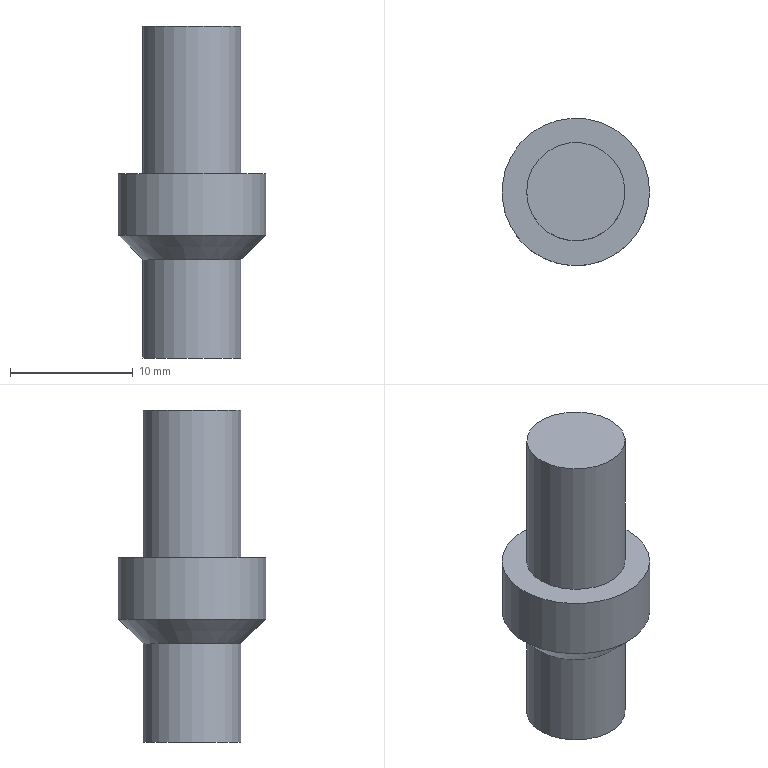Component | NX | PUNCH | 1 solid | 7 faces | box 12 x 12 x 27 mm | volume 1730 mm3 | plane 3 | cylinder 3 | cone 1 | commonest cylinder face diameters 8 x2 12 x1
STEP:
#1=CARTESIAN_POINT('',(0.,0.,0.));
#2=DIRECTION('',(0.,0.,1.));
#3=DIRECTION('',(1.,0.,0.));
#4=AXIS2_PLACEMENT_3D('',#1,#2,#3);
#5=CARTESIAN_POINT('',(11.5,0.,-25.997));
#6=VERTEX_POINT('',#5);
#7=CARTESIAN_POINT('',(7.5,0.,-25.997));
#8=DIRECTION('',(0.,0.,1.));
#9=DIRECTION('',(1.,0.,0.));
#10=AXIS2_PLACEMENT_3D('',#7,#8,#9);
#11=CIRCLE('',#10,4.);
#12=CARTESIAN_POINT('',(7.5,-4.,-25.997));
#13=DIRECTION('',(0.,0.,-1.));
#14=DIRECTION('',(-1.,0.,0.));
#15=AXIS2_PLACEMENT_3D('',#12,#13,#14);
#16=PLANE('',#15);
#17=CARTESIAN_POINT('',(-4.,4.));
#18=CARTESIAN_POINT('',(-4.,10.928));
#19=CARTESIAN_POINT('',(2.,7.464));
#20=CARTESIAN_POINT('',(8.,4.));
#21=CARTESIAN_POINT('',(2.,0.5359));
#22=CARTESIAN_POINT('',(-4.,-2.928));
#23=CARTESIAN_POINT('',(-4.,4.));
#24=(BOUNDED_CURVE()B_SPLINE_CURVE(2,(#17,#18,#19,#20,#21,#22,#23),.UNSPECIFIED.,.T.,.F.)B_SPLINE_CURVE_WITH_KNOTS((1,2,2,2,2,1),(-2.094,0.,2.094,4.189,6.283,8.378),.UNSPECIFIED.)CURVE()GEOMETRIC_REPRESENTATION_ITEM()RATIONAL_B_SPLINE_CURVE((1.,0.5,1.,0.5,1.,0.5,1.))REPRESENTATION_ITEM(''));
#25=(GEOMETRIC_REPRESENTATION_CONTEXT(2)PARAMETRIC_REPRESENTATION_CONTEXT()REPRESENTATION_CONTEXT('',''));
#26=DEFINITIONAL_REPRESENTATION('',(#24),#25);
#27=PCURVE('',#16,#26);
#28=CARTESIAN_POINT('',(7.5,0.,-25.997));
#29=DIRECTION('',(0.,0.,1.));
#30=DIRECTION('',(1.,0.,0.));
#31=AXIS2_PLACEMENT_3D('',#28,#29,#30);
#32=CYLINDRICAL_SURFACE('',#31,4.);
#33=CARTESIAN_POINT('',(0.,0.));
#34=DIRECTION('',(1.,0.));
#35=VECTOR('',#34,1.);
#36=LINE('',#33,#35);
#37=(GEOMETRIC_REPRESENTATION_CONTEXT(2)PARAMETRIC_REPRESENTATION_CONTEXT()REPRESENTATION_CONTEXT('',''));
#38=DEFINITIONAL_REPRESENTATION('',(#36),#37);
#39=PCURVE('',#32,#38);
#40=SURFACE_CURVE('',#11,(#27,#39),.PCURVE_S1.);
#41=EDGE_CURVE('',#6,#6,#40,.T.);
#42=ORIENTED_EDGE('',*,*,#41,.F.);
#43=EDGE_LOOP('',(#42));
#44=FACE_BOUND('',#43,.T.);
#45=ADVANCED_FACE('',(#44),#16,.T.);
#46=ORIENTED_EDGE('',*,*,#41,.T.);
#47=CARTESIAN_POINT('',(11.5,0.,-17.997));
#48=VERTEX_POINT('',#47);
#49=CARTESIAN_POINT('',(11.5,0.,-25.997));
#50=CARTESIAN_POINT('',(11.5,0.,-17.997));
#51=B_SPLINE_CURVE_WITH_KNOTS('',1,(#49,#50),.UNSPECIFIED.,.F.,.F.,(2,2),(0.,8.),.PIECEWISE_BEZIER_KNOTS.);
#52=CARTESIAN_POINT('',(6.283,0.));
#53=DIRECTION('',(0.,1.));
#54=VECTOR('',#53,1.);
#55=LINE('',#52,#54);
#56=(GEOMETRIC_REPRESENTATION_CONTEXT(2)PARAMETRIC_REPRESENTATION_CONTEXT()REPRESENTATION_CONTEXT('',''));
#57=DEFINITIONAL_REPRESENTATION('',(#55),#56);
#58=PCURVE('',#32,#57);
#59=CARTESIAN_POINT('',(0.,0.));
#60=DIRECTION('',(0.,1.));
#61=VECTOR('',#60,1.);
#62=LINE('',#59,#61);
#63=(GEOMETRIC_REPRESENTATION_CONTEXT(2)PARAMETRIC_REPRESENTATION_CONTEXT()REPRESENTATION_CONTEXT('',''));
#64=DEFINITIONAL_REPRESENTATION('',(#62),#63);
#65=PCURVE('',#32,#64);
#66=SEAM_CURVE('',#51,(#58,#65),.PCURVE_S1.);
#67=EDGE_CURVE('',#6,#48,#66,.T.);
#68=ORIENTED_EDGE('',*,*,#67,.T.);
#69=CARTESIAN_POINT('',(7.5,0.,-17.997));
#70=DIRECTION('',(0.,0.,1.));
#71=DIRECTION('',(1.,0.,0.));
#72=AXIS2_PLACEMENT_3D('',#69,#70,#71);
#73=CIRCLE('',#72,4.);
#74=CARTESIAN_POINT('',(0.,8.));
#75=DIRECTION('',(1.,0.));
#76=VECTOR('',#75,1.);
#77=LINE('',#74,#76);
#78=(GEOMETRIC_REPRESENTATION_CONTEXT(2)PARAMETRIC_REPRESENTATION_CONTEXT()REPRESENTATION_CONTEXT('',''));
#79=DEFINITIONAL_REPRESENTATION('',(#77),#78);
#80=PCURVE('',#32,#79);
#81=CARTESIAN_POINT('',(7.5,0.,-15.997));
#82=DIRECTION('',(0.,0.,1.));
#83=DIRECTION('',(1.,0.,0.));
#84=AXIS2_PLACEMENT_3D('',#81,#82,#83);
#85=CONICAL_SURFACE('',#84,6.,0.7854);
#86=CARTESIAN_POINT('',(0.,-2.));
#87=DIRECTION('',(1.,0.));
#88=VECTOR('',#87,1.);
#89=LINE('',#86,#88);
#90=(GEOMETRIC_REPRESENTATION_CONTEXT(2)PARAMETRIC_REPRESENTATION_CONTEXT()REPRESENTATION_CONTEXT('',''));
#91=DEFINITIONAL_REPRESENTATION('',(#89),#90);
#92=PCURVE('',#85,#91);
#93=SURFACE_CURVE('',#73,(#80,#92),.PCURVE_S1.);
#94=EDGE_CURVE('',#48,#48,#93,.T.);
#95=ORIENTED_EDGE('',*,*,#94,.F.);
#96=ORIENTED_EDGE('',*,*,#67,.F.);
#97=EDGE_LOOP('',(#46,#68,#95,#96));
#98=FACE_BOUND('',#97,.T.);
#99=ADVANCED_FACE('',(#98),#32,.T.);
#100=ORIENTED_EDGE('',*,*,#94,.T.);
#101=CARTESIAN_POINT('',(13.5,0.,-15.997));
#102=VERTEX_POINT('',#101);
#103=CARTESIAN_POINT('',(11.5,0.,-17.997));
#104=CARTESIAN_POINT('',(13.5,0.,-15.997));
#105=B_SPLINE_CURVE_WITH_KNOTS('',1,(#103,#104),.UNSPECIFIED.,.F.,.F.,(2,2),(-2.828,0.),.PIECEWISE_BEZIER_KNOTS.);
#106=CARTESIAN_POINT('',(6.283,0.));
#107=DIRECTION('',(0.,1.));
#108=VECTOR('',#107,1.);
#109=LINE('',#106,#108);
#110=(GEOMETRIC_REPRESENTATION_CONTEXT(2)PARAMETRIC_REPRESENTATION_CONTEXT()REPRESENTATION_CONTEXT('',''));
#111=DEFINITIONAL_REPRESENTATION('',(#109),#110);
#112=PCURVE('',#85,#111);
#113=CARTESIAN_POINT('',(0.,0.));
#114=DIRECTION('',(0.,1.));
#115=VECTOR('',#114,1.);
#116=LINE('',#113,#115);
#117=(GEOMETRIC_REPRESENTATION_CONTEXT(2)PARAMETRIC_REPRESENTATION_CONTEXT()REPRESENTATION_CONTEXT('',''));
#118=DEFINITIONAL_REPRESENTATION('',(#116),#117);
#119=PCURVE('',#85,#118);
#120=SEAM_CURVE('',#105,(#112,#119),.PCURVE_S1.);
#121=EDGE_CURVE('',#48,#102,#120,.T.);
#122=ORIENTED_EDGE('',*,*,#121,.T.);
#123=CARTESIAN_POINT('',(7.5,0.,-15.997));
#124=DIRECTION('',(0.,0.,1.));
#125=DIRECTION('',(1.,0.,0.));
#126=AXIS2_PLACEMENT_3D('',#123,#124,#125);
#127=CIRCLE('',#126,6.);
#128=CARTESIAN_POINT('',(0.,0.));
#129=DIRECTION('',(1.,0.));
#130=VECTOR('',#129,1.);
#131=LINE('',#128,#130);
#132=(GEOMETRIC_REPRESENTATION_CONTEXT(2)PARAMETRIC_REPRESENTATION_CONTEXT()REPRESENTATION_CONTEXT('',''));
#133=DEFINITIONAL_REPRESENTATION('',(#131),#132);
#134=PCURVE('',#85,#133);
#135=CARTESIAN_POINT('',(7.5,0.,-25.997));
#136=DIRECTION('',(0.,0.,1.));
#137=DIRECTION('',(1.,0.,0.));
#138=AXIS2_PLACEMENT_3D('',#135,#136,#137);
#139=CYLINDRICAL_SURFACE('',#138,6.);
#140=CARTESIAN_POINT('',(0.,10.));
#141=DIRECTION('',(1.,0.));
#142=VECTOR('',#141,1.);
#143=LINE('',#140,#142);
#144=(GEOMETRIC_REPRESENTATION_CONTEXT(2)PARAMETRIC_REPRESENTATION_CONTEXT()REPRESENTATION_CONTEXT('',''));
#145=DEFINITIONAL_REPRESENTATION('',(#143),#144);
#146=PCURVE('',#139,#145);
#147=SURFACE_CURVE('',#127,(#134,#146),.PCURVE_S1.);
#148=EDGE_CURVE('',#102,#102,#147,.T.);
#149=ORIENTED_EDGE('',*,*,#148,.F.);
#150=ORIENTED_EDGE('',*,*,#121,.F.);
#151=EDGE_LOOP('',(#100,#122,#149,#150));
#152=FACE_BOUND('',#151,.T.);
#153=ADVANCED_FACE('',(#152),#85,.T.);
#154=ORIENTED_EDGE('',*,*,#148,.T.);
#155=CARTESIAN_POINT('',(13.5,0.,-10.997));
#156=VERTEX_POINT('',#155);
#157=CARTESIAN_POINT('',(13.5,0.,-15.997));
#158=CARTESIAN_POINT('',(13.5,0.,-10.997));
#159=B_SPLINE_CURVE_WITH_KNOTS('',1,(#157,#158),.UNSPECIFIED.,.F.,.F.,(2,2),(10.,15.),.PIECEWISE_BEZIER_KNOTS.);
#160=CARTESIAN_POINT('',(6.283,0.));
#161=DIRECTION('',(0.,1.));
#162=VECTOR('',#161,1.);
#163=LINE('',#160,#162);
#164=(GEOMETRIC_REPRESENTATION_CONTEXT(2)PARAMETRIC_REPRESENTATION_CONTEXT()REPRESENTATION_CONTEXT('',''));
#165=DEFINITIONAL_REPRESENTATION('',(#163),#164);
#166=PCURVE('',#139,#165);
#167=CARTESIAN_POINT('',(0.,0.));
#168=DIRECTION('',(0.,1.));
#169=VECTOR('',#168,1.);
#170=LINE('',#167,#169);
#171=(GEOMETRIC_REPRESENTATION_CONTEXT(2)PARAMETRIC_REPRESENTATION_CONTEXT()REPRESENTATION_CONTEXT('',''));
#172=DEFINITIONAL_REPRESENTATION('',(#170),#171);
#173=PCURVE('',#139,#172);
#174=SEAM_CURVE('',#159,(#166,#173),.PCURVE_S1.);
#175=EDGE_CURVE('',#102,#156,#174,.T.);
#176=ORIENTED_EDGE('',*,*,#175,.T.);
#177=CARTESIAN_POINT('',(7.5,0.,-10.997));
#178=DIRECTION('',(0.,0.,1.));
#179=DIRECTION('',(1.,0.,0.));
#180=AXIS2_PLACEMENT_3D('',#177,#178,#179);
#181=CIRCLE('',#180,6.);
#182=CARTESIAN_POINT('',(0.,15.));
#183=DIRECTION('',(1.,0.));
#184=VECTOR('',#183,1.);
#185=LINE('',#182,#184);
#186=(GEOMETRIC_REPRESENTATION_CONTEXT(2)PARAMETRIC_REPRESENTATION_CONTEXT()REPRESENTATION_CONTEXT('',''));
#187=DEFINITIONAL_REPRESENTATION('',(#185),#186);
#188=PCURVE('',#139,#187);
#189=CARTESIAN_POINT('',(7.5,-4.,-10.997));
#190=DIRECTION('',(0.,0.,1.));
#191=DIRECTION('',(1.,0.,0.));
#192=AXIS2_PLACEMENT_3D('',#189,#190,#191);
#193=PLANE('',#192);
#194=CARTESIAN_POINT('',(0.,4.));
#195=DIRECTION('',(1.,0.));
#196=AXIS2_PLACEMENT_2D('',#194,#195);
#197=CIRCLE('',#196,6.);
#198=(GEOMETRIC_REPRESENTATION_CONTEXT(2)PARAMETRIC_REPRESENTATION_CONTEXT()REPRESENTATION_CONTEXT('',''));
#199=DEFINITIONAL_REPRESENTATION('',(#197),#198);
#200=PCURVE('',#193,#199);
#201=SURFACE_CURVE('',#181,(#188,#200),.PCURVE_S1.);
#202=EDGE_CURVE('',#156,#156,#201,.T.);
#203=ORIENTED_EDGE('',*,*,#202,.F.);
#204=ORIENTED_EDGE('',*,*,#175,.F.);
#205=EDGE_LOOP('',(#154,#176,#203,#204));
#206=FACE_BOUND('',#205,.T.);
#207=ADVANCED_FACE('',(#206),#139,.T.);
#208=ORIENTED_EDGE('',*,*,#202,.T.);
#209=EDGE_LOOP('',(#208));
#210=FACE_BOUND('',#209,.T.);
#211=CARTESIAN_POINT('',(11.5,0.,-10.997));
#212=VERTEX_POINT('',#211);
#213=CARTESIAN_POINT('',(7.5,0.,-10.997));
#214=DIRECTION('',(0.,0.,1.));
#215=DIRECTION('',(1.,0.,0.));
#216=AXIS2_PLACEMENT_3D('',#213,#214,#215);
#217=CIRCLE('',#216,4.);
#218=CARTESIAN_POINT('',(0.,4.));
#219=DIRECTION('',(1.,0.));
#220=AXIS2_PLACEMENT_2D('',#218,#219);
#221=CIRCLE('',#220,4.);
#222=(GEOMETRIC_REPRESENTATION_CONTEXT(2)PARAMETRIC_REPRESENTATION_CONTEXT()REPRESENTATION_CONTEXT('',''));
#223=DEFINITIONAL_REPRESENTATION('',(#221),#222);
#224=PCURVE('',#193,#223);
#225=CARTESIAN_POINT('',(7.5,0.,-25.997));
#226=DIRECTION('',(0.,0.,1.));
#227=DIRECTION('',(1.,0.,0.));
#228=AXIS2_PLACEMENT_3D('',#225,#226,#227);
#229=CYLINDRICAL_SURFACE('',#228,4.);
#230=CARTESIAN_POINT('',(0.,15.));
#231=DIRECTION('',(1.,0.));
#232=VECTOR('',#231,1.);
#233=LINE('',#230,#232);
#234=(GEOMETRIC_REPRESENTATION_CONTEXT(2)PARAMETRIC_REPRESENTATION_CONTEXT()REPRESENTATION_CONTEXT('',''));
#235=DEFINITIONAL_REPRESENTATION('',(#233),#234);
#236=PCURVE('',#229,#235);
#237=SURFACE_CURVE('',#217,(#224,#236),.PCURVE_S1.);
#238=EDGE_CURVE('',#212,#212,#237,.T.);
#239=ORIENTED_EDGE('',*,*,#238,.F.);
#240=EDGE_LOOP('',(#239));
#241=FACE_BOUND('',#240,.T.);
#242=ADVANCED_FACE('',(#210,#241),#193,.T.);
#243=ORIENTED_EDGE('',*,*,#238,.T.);
#244=CARTESIAN_POINT('',(11.5,0.,1.003));
#245=VERTEX_POINT('',#244);
#246=CARTESIAN_POINT('',(11.5,0.,-10.997));
#247=CARTESIAN_POINT('',(11.5,0.,1.003));
#248=B_SPLINE_CURVE_WITH_KNOTS('',1,(#246,#247),.UNSPECIFIED.,.F.,.F.,(2,2),(15.,27.),.PIECEWISE_BEZIER_KNOTS.);
#249=CARTESIAN_POINT('',(6.283,0.));
#250=DIRECTION('',(0.,1.));
#251=VECTOR('',#250,1.);
#252=LINE('',#249,#251);
#253=(GEOMETRIC_REPRESENTATION_CONTEXT(2)PARAMETRIC_REPRESENTATION_CONTEXT()REPRESENTATION_CONTEXT('',''));
#254=DEFINITIONAL_REPRESENTATION('',(#252),#253);
#255=PCURVE('',#229,#254);
#256=CARTESIAN_POINT('',(0.,0.));
#257=DIRECTION('',(0.,1.));
#258=VECTOR('',#257,1.);
#259=LINE('',#256,#258);
#260=(GEOMETRIC_REPRESENTATION_CONTEXT(2)PARAMETRIC_REPRESENTATION_CONTEXT()REPRESENTATION_CONTEXT('',''));
#261=DEFINITIONAL_REPRESENTATION('',(#259),#260);
#262=PCURVE('',#229,#261);
#263=SEAM_CURVE('',#248,(#255,#262),.PCURVE_S1.);
#264=EDGE_CURVE('',#212,#245,#263,.T.);
#265=ORIENTED_EDGE('',*,*,#264,.T.);
#266=CARTESIAN_POINT('',(7.5,0.,1.003));
#267=DIRECTION('',(0.,0.,1.));
#268=DIRECTION('',(1.,0.,0.));
#269=AXIS2_PLACEMENT_3D('',#266,#267,#268);
#270=CIRCLE('',#269,4.);
#271=CARTESIAN_POINT('',(0.,27.));
#272=DIRECTION('',(1.,0.));
#273=VECTOR('',#272,1.);
#274=LINE('',#271,#273);
#275=(GEOMETRIC_REPRESENTATION_CONTEXT(2)PARAMETRIC_REPRESENTATION_CONTEXT()REPRESENTATION_CONTEXT('',''));
#276=DEFINITIONAL_REPRESENTATION('',(#274),#275);
#277=PCURVE('',#229,#276);
#278=CARTESIAN_POINT('',(7.5,0.,1.003));
#279=DIRECTION('',(0.,0.,1.));
#280=DIRECTION('',(1.,0.,0.));
#281=AXIS2_PLACEMENT_3D('',#278,#279,#280);
#282=PLANE('',#281);
#283=CARTESIAN_POINT('',(0.,0.));
#284=DIRECTION('',(1.,0.));
#285=AXIS2_PLACEMENT_2D('',#283,#284);
#286=CIRCLE('',#285,4.);
#287=(GEOMETRIC_REPRESENTATION_CONTEXT(2)PARAMETRIC_REPRESENTATION_CONTEXT()REPRESENTATION_CONTEXT('',''));
#288=DEFINITIONAL_REPRESENTATION('',(#286),#287);
#289=PCURVE('',#282,#288);
#290=SURFACE_CURVE('',#270,(#277,#289),.PCURVE_S1.);
#291=EDGE_CURVE('',#245,#245,#290,.T.);
#292=ORIENTED_EDGE('',*,*,#291,.F.);
#293=ORIENTED_EDGE('',*,*,#264,.F.);
#294=EDGE_LOOP('',(#243,#265,#292,#293));
#295=FACE_BOUND('',#294,.T.);
#296=ADVANCED_FACE('',(#295),#229,.T.);
#297=ORIENTED_EDGE('',*,*,#291,.T.);
#298=EDGE_LOOP('',(#297));
#299=FACE_BOUND('',#298,.T.);
#300=ADVANCED_FACE('',(#299),#282,.T.);
#301=CLOSED_SHELL('',(#45,#99,#153,#207,#242,#296,#300));
#302=MANIFOLD_SOLID_BREP('',#301);
#303=(LENGTH_UNIT()NAMED_UNIT(*)SI_UNIT(.MILLI.,.METRE.));
#304=UNCERTAINTY_MEASURE_WITH_UNIT(LENGTH_MEASURE(0.00001),#303,'','');
#305=(NAMED_UNIT(*)PLANE_ANGLE_UNIT()SI_UNIT($,.RADIAN.));
#306=(NAMED_UNIT(*)SI_UNIT($,.STERADIAN.)SOLID_ANGLE_UNIT());
#307=(GEOMETRIC_REPRESENTATION_CONTEXT(3)GLOBAL_UNCERTAINTY_ASSIGNED_CONTEXT((#304))GLOBAL_UNIT_ASSIGNED_CONTEXT((#303,#305,#306))REPRESENTATION_CONTEXT('',''));
#308=ADVANCED_BREP_SHAPE_REPRESENTATION('',(#4,#302),#307);